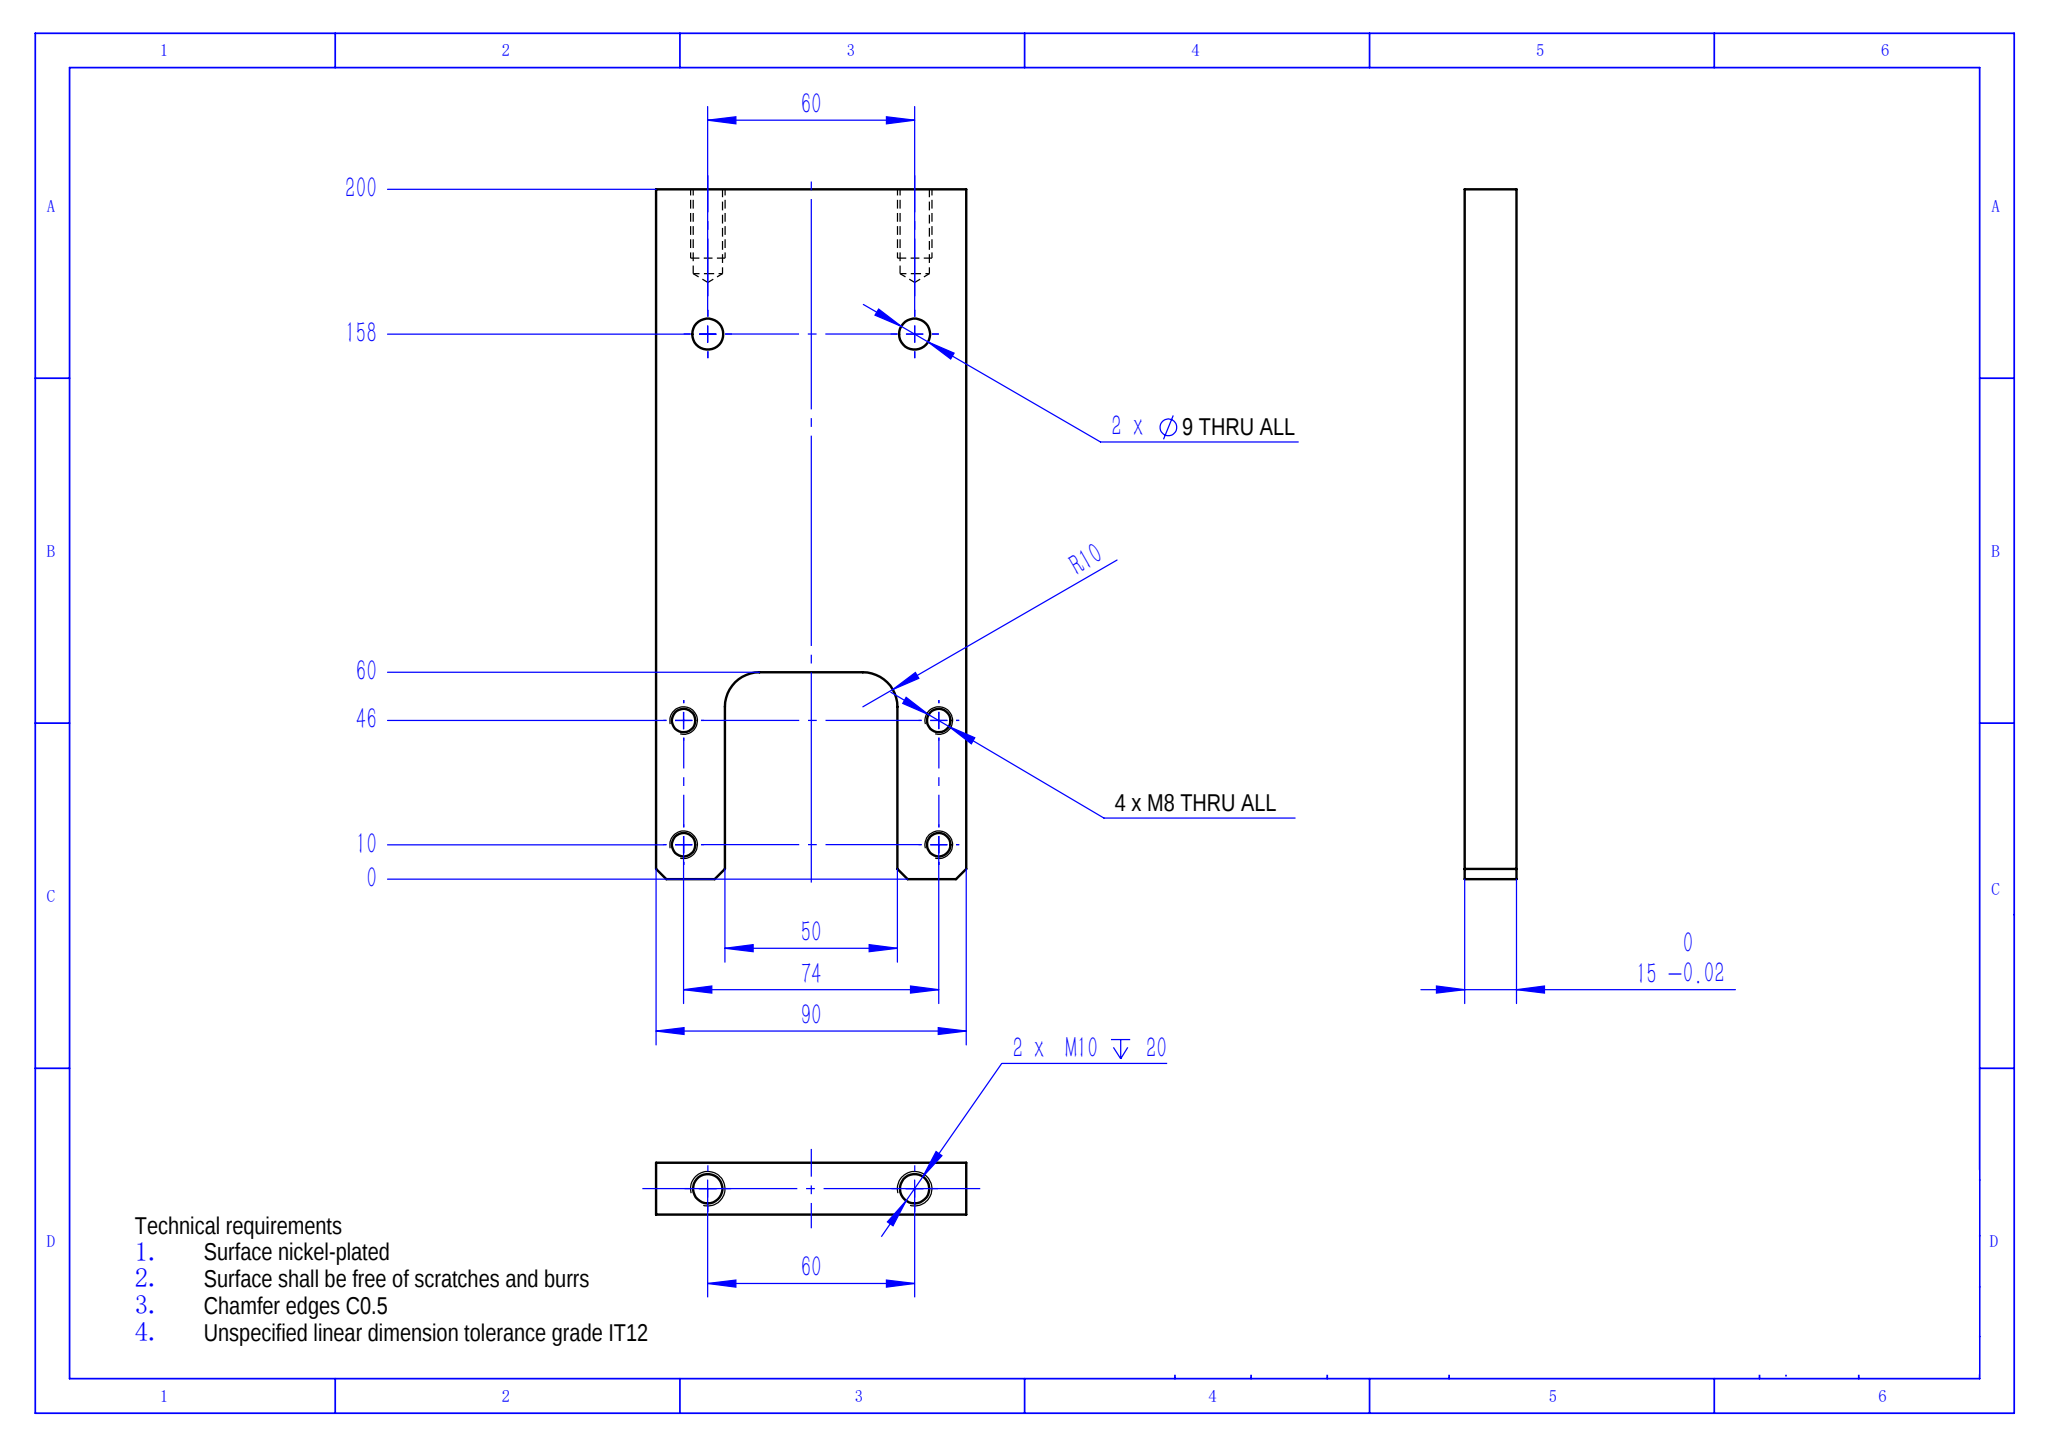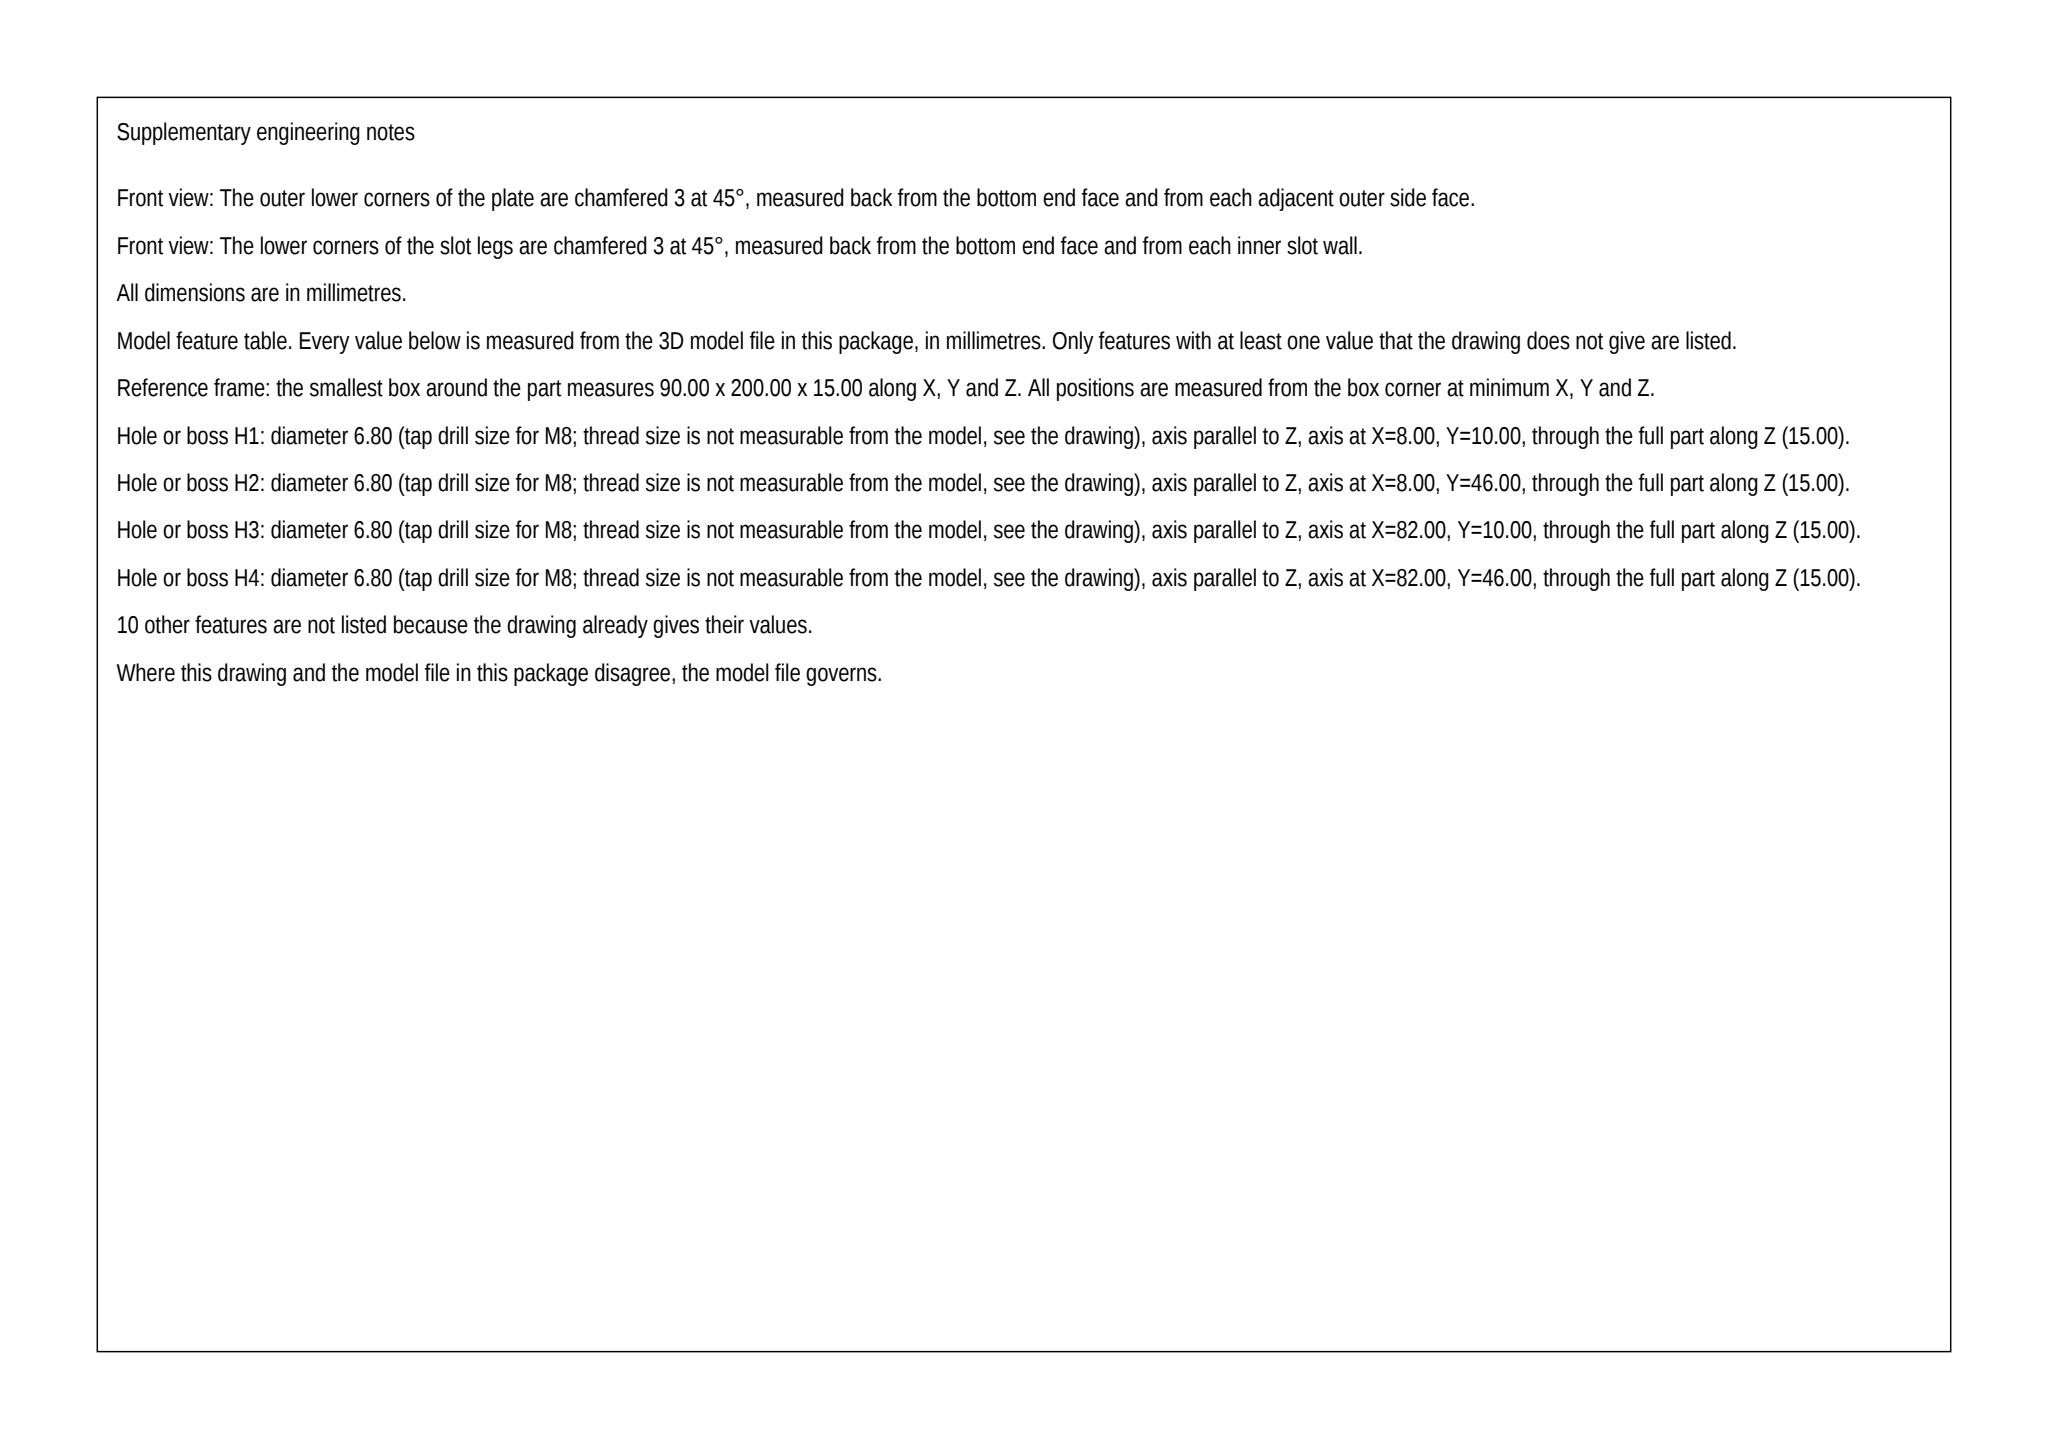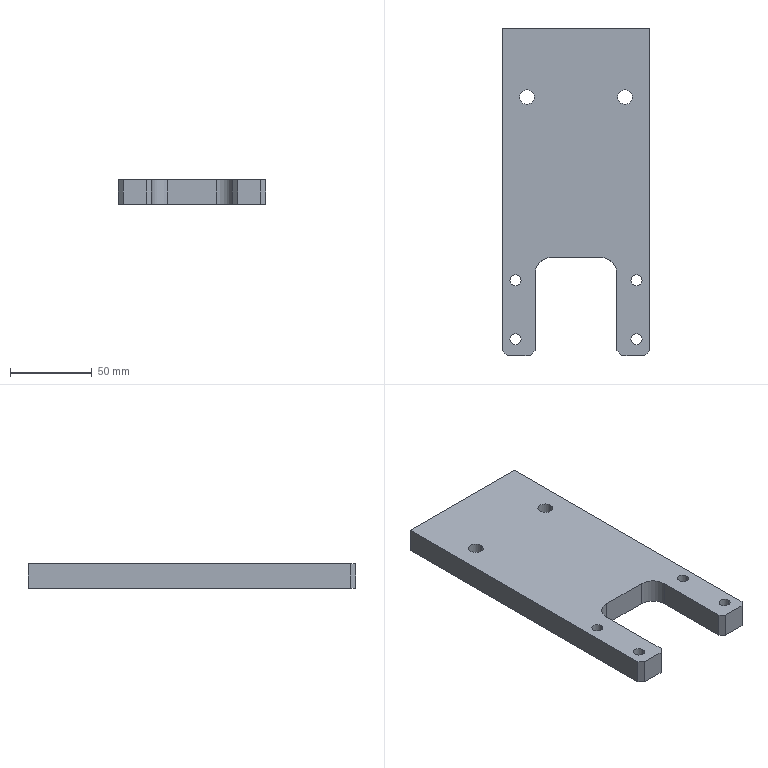Part | SolidWorks | mm | 1 solid | 36 faces | box 90 x 200 x 15 mm | volume 218409 mm3 | cylinder 18 | plane 14 | cone 4 | commonest cylinder face diameters 6.8 x8 9 x4 8.5 x4 20 x2
build123d program:
from build123d import *

# Parameters (mm, degrees)
SKETCH1_W              = 90
SKETCH1_H              = 200
BOSS_EXTRUDE1_DEPTH    = 7.5
M10_TAPPED_HOLE1_D     = 8.5
M10_TAPPED_HOLE1_DEPTH = 24.5
M10_TAPPED_HOLE1_TIP   = 2.554
M8_TAPPED_HOLE1_D      = 6.8
CUT_EXTRUDE1_DEPTH     = 206.548
CHAMFER1_SIZE          = 3
M8_CLEARANCE_HOLE2_D   = 9


with BuildPart() as part:
    # Sketch1 → Boss-Extrude1 (new, symmetric)
    with BuildSketch(Plane.XY):
        with Locations((0, -100)):
            Rectangle(SKETCH1_W, SKETCH1_H)
    extrude(amount=BOSS_EXTRUDE1_DEPTH, both=True)

    # M10 Tapped Hole1
    with Locations(Plane(origin=(0, 0, 0), x_dir=(1, 0, 0), z_dir=(0, 1, 0))):
        with Locations((-30, 0), (30, 0)):
            Hole(M10_TAPPED_HOLE1_D / 2, depth=M10_TAPPED_HOLE1_DEPTH)
            with Locations((0, 0, -(M10_TAPPED_HOLE1_DEPTH + M10_TAPPED_HOLE1_TIP / 2))):  # 118° drill point
                Cone(0, M10_TAPPED_HOLE1_D / 2, M10_TAPPED_HOLE1_TIP, mode=Mode.SUBTRACT)

    # M8 Tapped Hole1 (through all)
    with Locations(Plane.XY.offset(7.5)):
        with Locations((-37, -154), (-37, -190), (37, -154), (37, -190)):
            Hole(M8_TAPPED_HOLE1_D / 2)

    # Sketch6 → Cut-Extrude1 (cut, through all)
    with BuildSketch(Plane.XY.offset(7.5)):
        with BuildLine():
            Line((-25, -200), (25, -200))
            Line((25, -200), (25, -150))
            ThreePointArc((25, -150), (22.071, -142.929), (15, -140))
            Line((15, -140), (-15, -140))
            ThreePointArc((-15, -140), (-22.071, -142.929), (-25, -150))
            Line((-25, -150), (-25, -200))
        make_face()
    extrude(amount=-CUT_EXTRUDE1_DEPTH, mode=Mode.SUBTRACT)

    # Chamfer1
    chamfer1_edges = [part.edges().sort_by_distance(p)[0] for p in [
        (-25, -200, 0),
        (25, -200, 0),
        (45, -200, 0),
        (-45, -200, 0),
    ]]
    chamfer(chamfer1_edges, length=CHAMFER1_SIZE)

    # M8 Clearance Hole2 (through all)
    with Locations(Plane(origin=(0, 0, -7.5), x_dir=(-1, 0, 0), z_dir=(0, 0, -1))):
        with Locations((-30, -42), (30, -42)):
            Hole(M8_CLEARANCE_HOLE2_D / 2)


solid = part.part